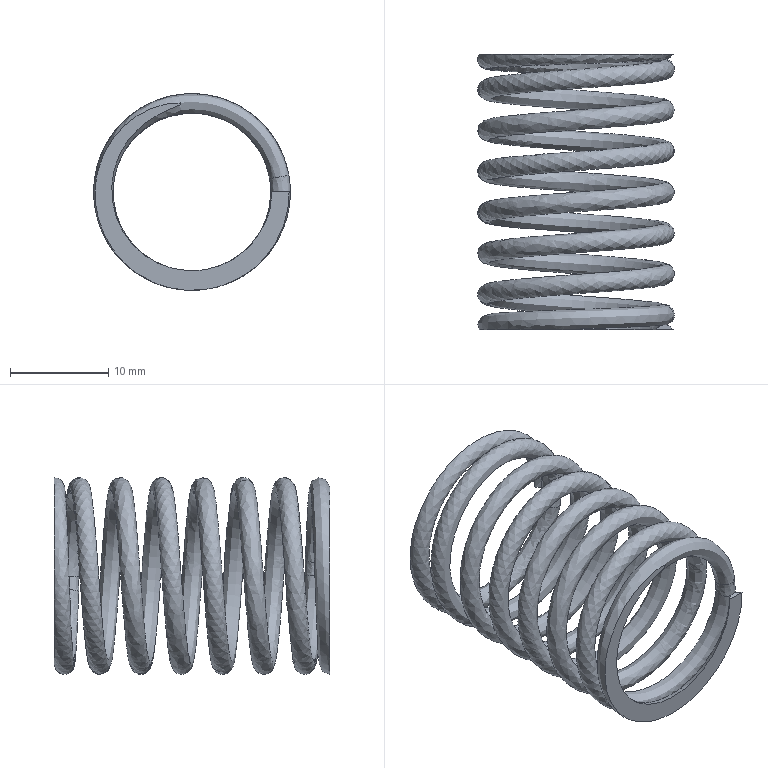Component | NX | SPRING | 1 solid | 9 faces | volume 1307 mm3 | spline 5 | plane 4